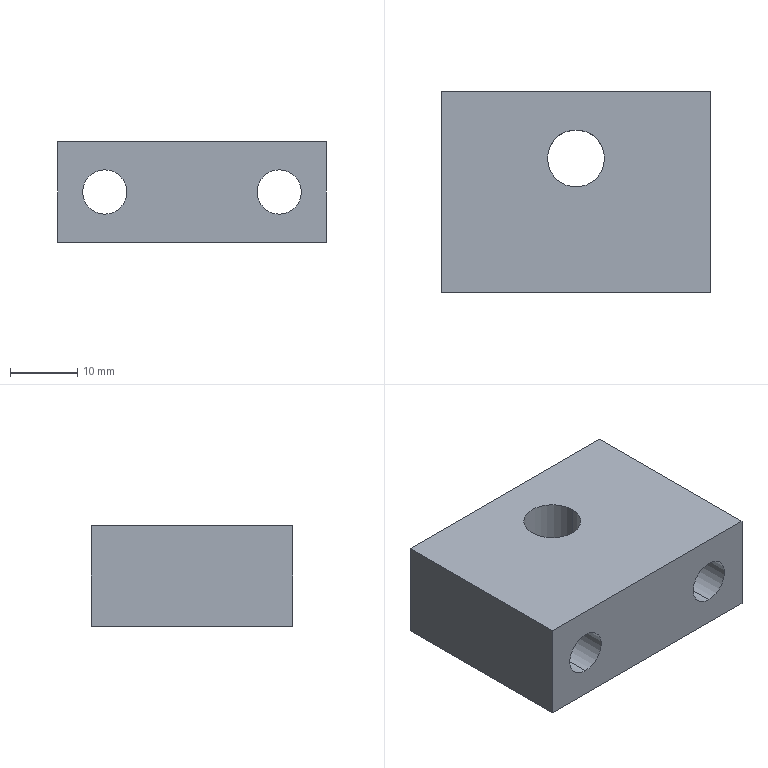CAM job | Mastercam | mm | 11 operations | part box 40 x 35 x 15
1. Facing | 24 - 100 平铣刀
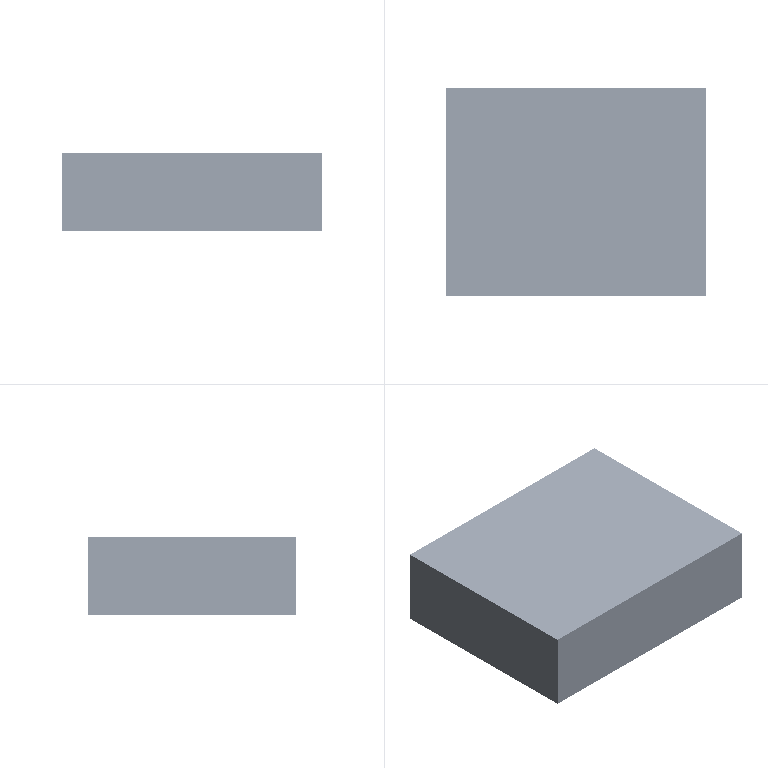2. Contour (Ramp) | 9 - 10 平铣刀
3. Contour (2D) | 10 - 10 平铣刀
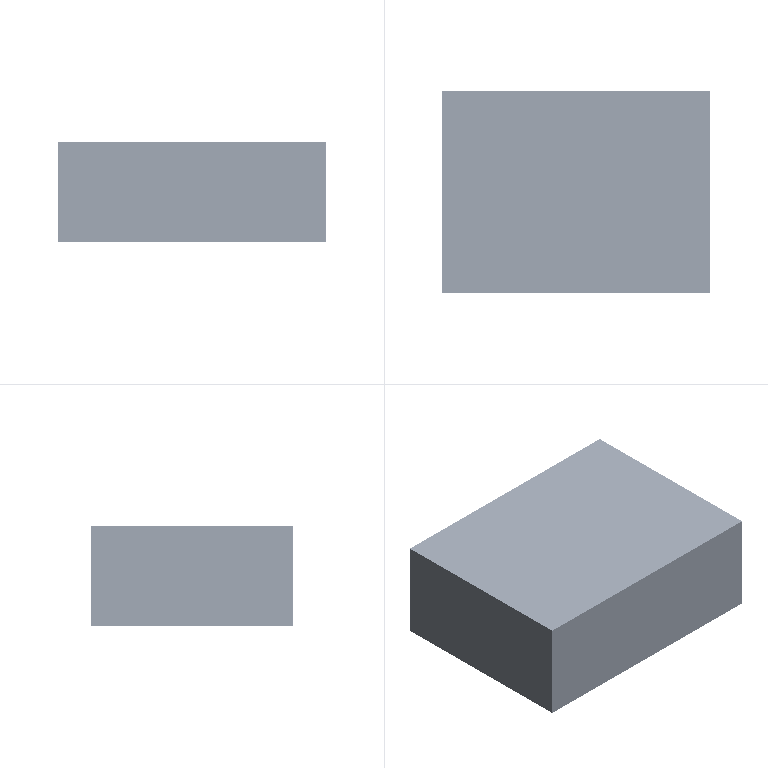4. Drill/Counterbore | 7 - 4 倒角刀
5. Contour (2D chamfer) | 7 - 4 倒角刀
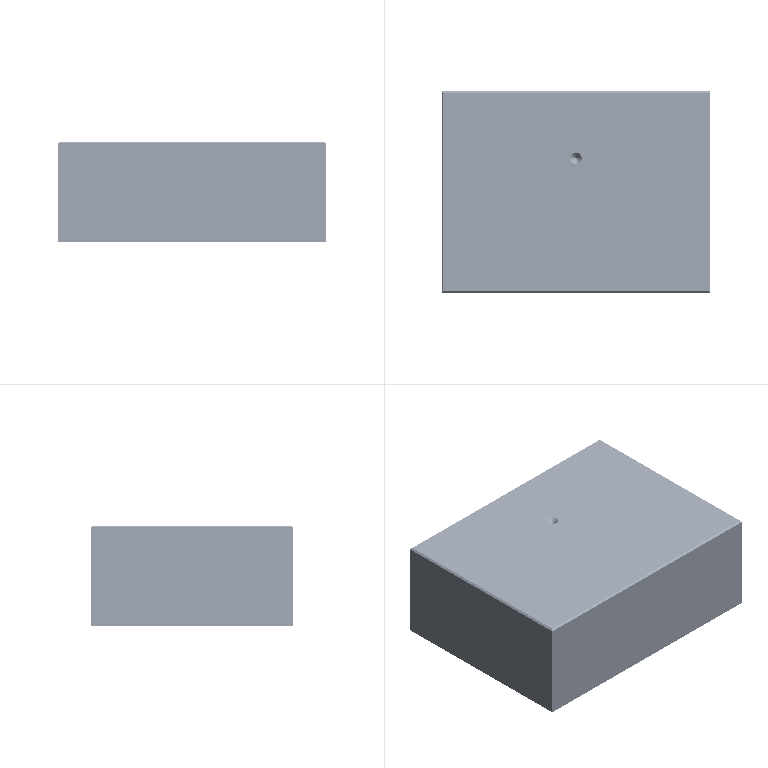6. Facing | 24 - 100 平铣刀
7. Contour (2D chamfer) | 7 - 4 倒角刀
8. Contour (Ramp) | 6 - 6 平铣刀
9. Contour (2D) | 6 - 6 平铣刀
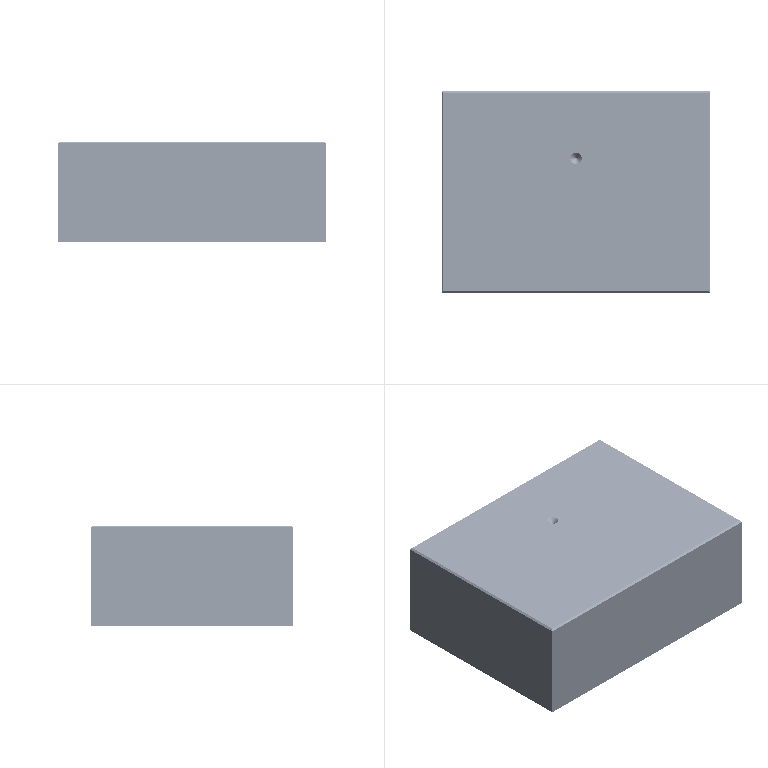10. Drill/Counterbore | 7 - 4 倒角刀
11. Contour (2D chamfer) | 7 - 4 倒角刀